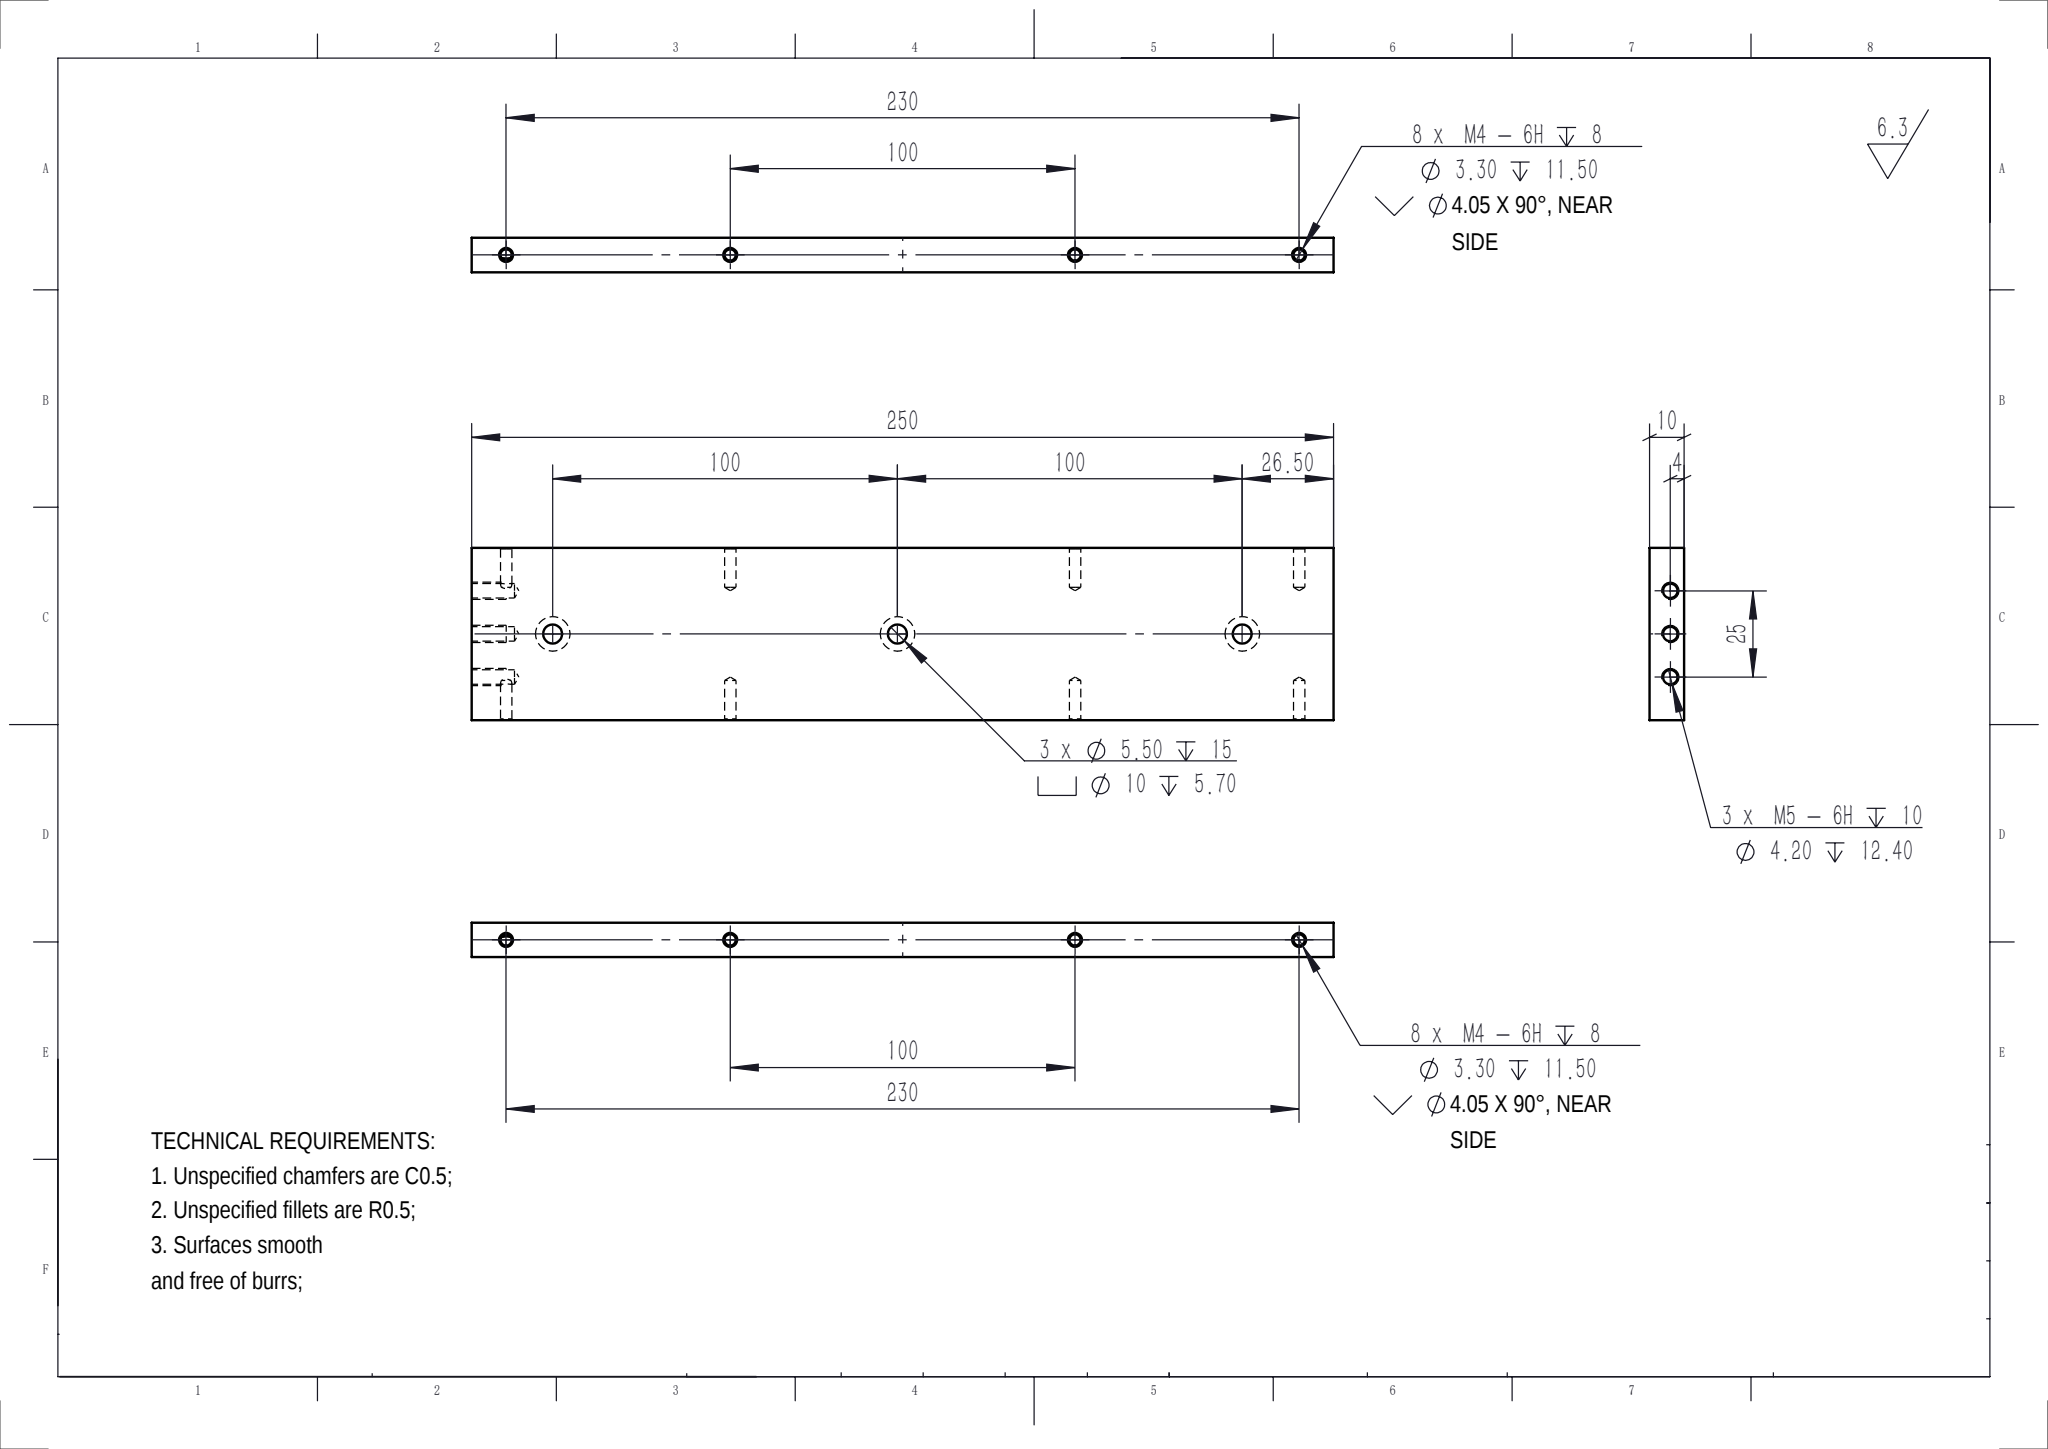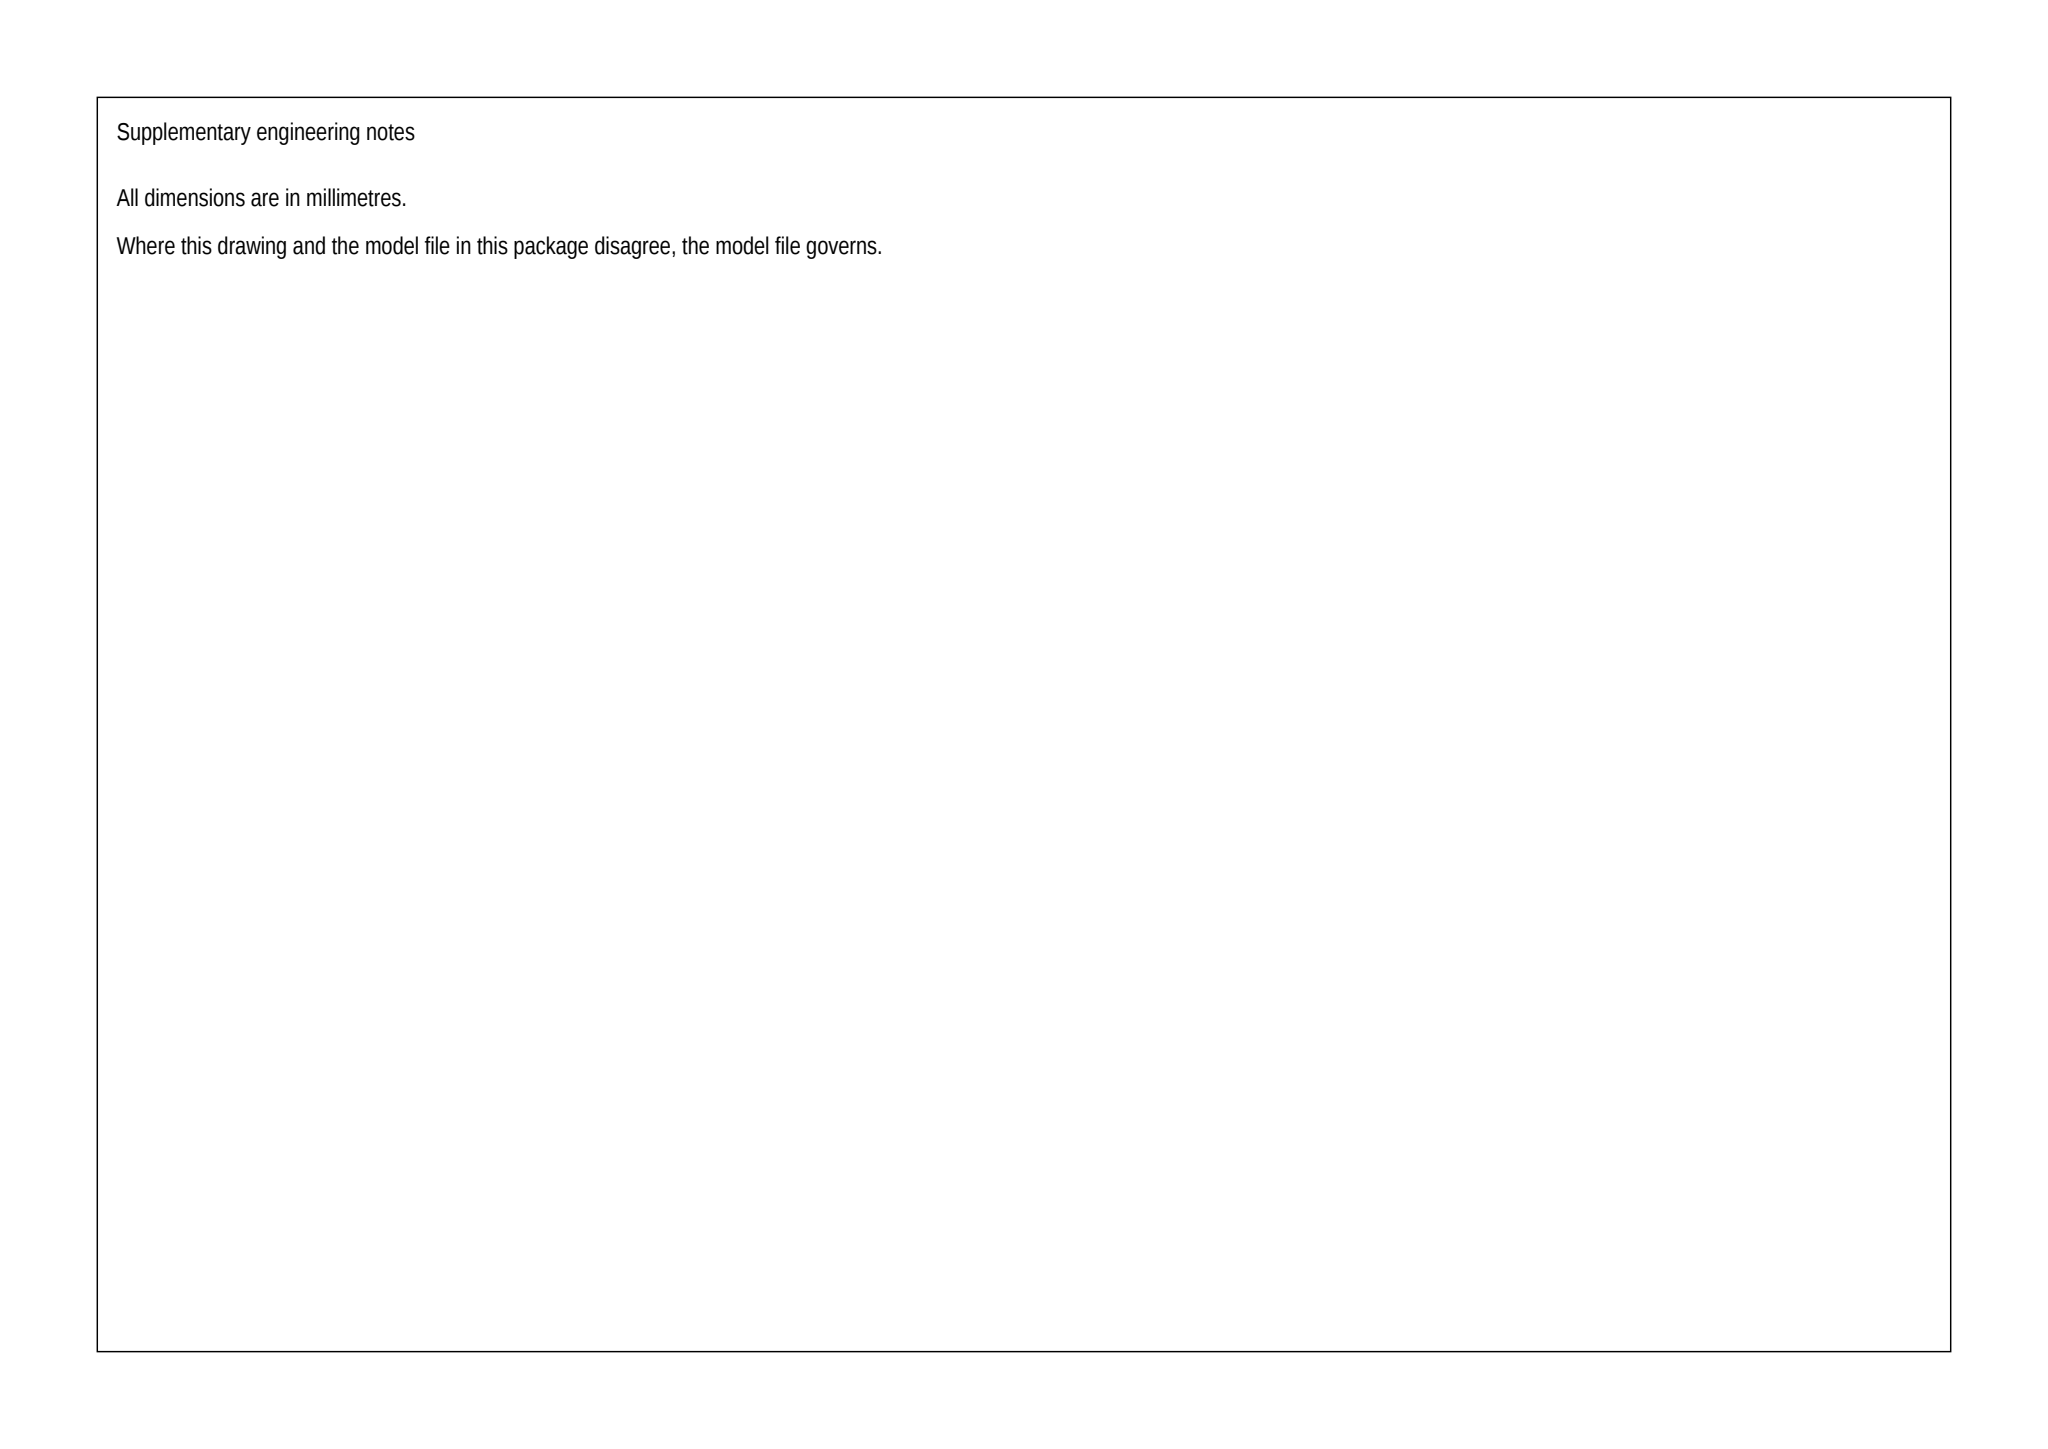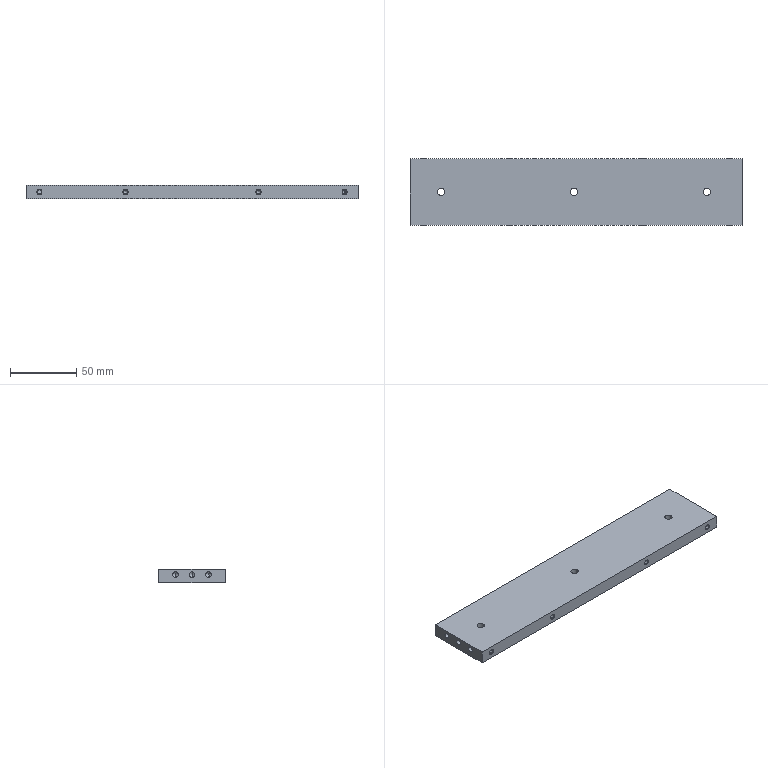Part | SolidWorks | mm | 1 solid | 80 faces | box 250 x 50 x 10 mm | volume 122019 mm3 | cone 37 | cylinder 34 | plane 9 | commonest cylinder face diameters 3.3 x16 4.2 x6 10 x6 5.5 x6
build123d program:
from build123d import *

# Parameters (mm, degrees)
SKETCH1_W                                         = 250
SKETCH1_H                                         = 50
BOSS_EXTRUDE1_DEPTH                               = 10
M4_TAPPED_HOLE1_AT_2_COUNT                        = 2
M4_TAPPED_HOLE1_AT_2_PITCH                        = 65
M4_TAPPED_HOLE1_AT_3_COUNT                        = 2
M4_TAPPED_HOLE1_AT_3_PITCH                        = 165
M4_TAPPED_HOLE1_AT_4_COUNT                        = 2
M4_TAPPED_HOLE1_AT_4_PITCH                        = 230
HOLE_SIZE_ACCORDING_TO_HEXAGON_SOCKET_D           = 5.5
HOLE_SIZE_ACCORDING_TO_HEXAGON_SOCKET_DEPTH       = 15
HOLE_SIZE_ACCORDING_TO_HEXAGON_SOCKET_CBORE_D     = 10
HOLE_SIZE_ACCORDING_TO_HEXAGON_SOCKET_CBORE_DEPTH = 5.7
HOLE_SIZE_ACCORDING_TO_HEXAGON_SOCKET_TIP         = 1.652
M5_TAPPED_HOLE1_D                                 = 4.2
M5_TAPPED_HOLE1_DEPTH                             = 12.4
M5_TAPPED_HOLE1_TIP                               = 1.262


with BuildPart() as part:
    # Sketch1 → Boss-Extrude1 (new body)
    with BuildSketch(Plane.XY):
        Rectangle(SKETCH1_W, SKETCH1_H)
    extrude(amount=BOSS_EXTRUDE1_DEPTH)

    # Sketch3 → M4 Tapped Hole1 (revolve, cut)
    with BuildSketch(Plane(origin=(-115, -25, 5), x_dir=(0, 0, -1), z_dir=(1, 0, 0))):
        Polygon((0, 0), (0, 12.491), (1.65, 11.5), (1.65, 0.375), (2.025, 0), align=None)
    m4_tapped_hole1 = revolve(axis=Axis((-115, -31.35, 5), (0, 1, 0)), mode=Mode.SUBTRACT)

    # M4 Tapped Hole1 at 2: M4 Tapped Hole1 ×2
    with Locations(*[(i * M4_TAPPED_HOLE1_AT_2_PITCH, 0, 0) for i in range(1, M4_TAPPED_HOLE1_AT_2_COUNT)]):
        add(m4_tapped_hole1, mode=Mode.SUBTRACT)

    # M4 Tapped Hole1 at 3: M4 Tapped Hole1 ×2
    with Locations(*[(i * M4_TAPPED_HOLE1_AT_3_PITCH, 0, 0) for i in range(1, M4_TAPPED_HOLE1_AT_3_COUNT)]):
        add(m4_tapped_hole1, mode=Mode.SUBTRACT)

    # M4 Tapped Hole1 at 4: M4 Tapped Hole1 ×2
    with Locations(*[(i * M4_TAPPED_HOLE1_AT_4_PITCH, 0, 0) for i in range(1, M4_TAPPED_HOLE1_AT_4_COUNT)]):
        add(m4_tapped_hole1, mode=Mode.SUBTRACT)

    # Mirror1: M4 Tapped Hole1 across plane
    add(m4_tapped_hole1.mirror(Plane.ZX), mode=Mode.SUBTRACT)

    # Mirror1 copy 1 sketch → Mirror1 copy 1 (revolve, cut)
    with BuildSketch(Plane(origin=(-50, 25, 5), x_dir=(0, 0, -1), z_dir=(1, 0, 0))):
        Polygon((0, 0), (0, -12.491), (1.65, -11.5), (1.65, -0.375), (2.025, 0), align=None)
    revolve(axis=Axis((-50, 31.35, 5), (0, 1, 0)), mode=Mode.SUBTRACT)

    # Mirror1 copy 2 sketch → Mirror1 copy 2 (revolve, cut)
    with BuildSketch(Plane(origin=(50, 25, 5), x_dir=(0, 0, -1), z_dir=(1, 0, 0))):
        Polygon((0, 0), (0, -12.491), (1.65, -11.5), (1.65, -0.375), (2.025, 0), align=None)
    revolve(axis=Axis((50, 31.35, 5), (0, 1, 0)), mode=Mode.SUBTRACT)

    # Mirror1 copy 3 sketch → Mirror1 copy 3 (revolve, cut)
    with BuildSketch(Plane(origin=(115, 25, 5), x_dir=(0, 0, -1), z_dir=(1, 0, 0))):
        Polygon((0, 0), (0, -12.491), (1.65, -11.5), (1.65, -0.375), (2.025, 0), align=None)
    revolve(axis=Axis((115, 31.35, 5), (0, 1, 0)), mode=Mode.SUBTRACT)

    # Hole Size _ according to_ Hexagon Socket
    with Locations(Plane(origin=(0, 0, 0), x_dir=(-1, 0, 0), z_dir=(0, 0, -1))):
        with Locations((101.5, 0), (1.5, 0), (-98.5, 0)):
            CounterBoreHole(HOLE_SIZE_ACCORDING_TO_HEXAGON_SOCKET_D / 2, HOLE_SIZE_ACCORDING_TO_HEXAGON_SOCKET_CBORE_D / 2, HOLE_SIZE_ACCORDING_TO_HEXAGON_SOCKET_CBORE_DEPTH, depth=HOLE_SIZE_ACCORDING_TO_HEXAGON_SOCKET_DEPTH)
            with Locations((0, 0, -(HOLE_SIZE_ACCORDING_TO_HEXAGON_SOCKET_DEPTH + HOLE_SIZE_ACCORDING_TO_HEXAGON_SOCKET_TIP / 2))):  # 118° drill point
                Cone(0, HOLE_SIZE_ACCORDING_TO_HEXAGON_SOCKET_D / 2, HOLE_SIZE_ACCORDING_TO_HEXAGON_SOCKET_TIP, mode=Mode.SUBTRACT)

    # M5 Tapped Hole1
    with Locations(Plane.ZY.offset(125)):
        with Locations((6, 12.5), (6, 0), (6, -12.5)):
            Hole(M5_TAPPED_HOLE1_D / 2, depth=M5_TAPPED_HOLE1_DEPTH)
            with Locations((0, 0, -(M5_TAPPED_HOLE1_DEPTH + M5_TAPPED_HOLE1_TIP / 2))):  # 118° drill point
                Cone(0, M5_TAPPED_HOLE1_D / 2, M5_TAPPED_HOLE1_TIP, mode=Mode.SUBTRACT)


solid = part.part